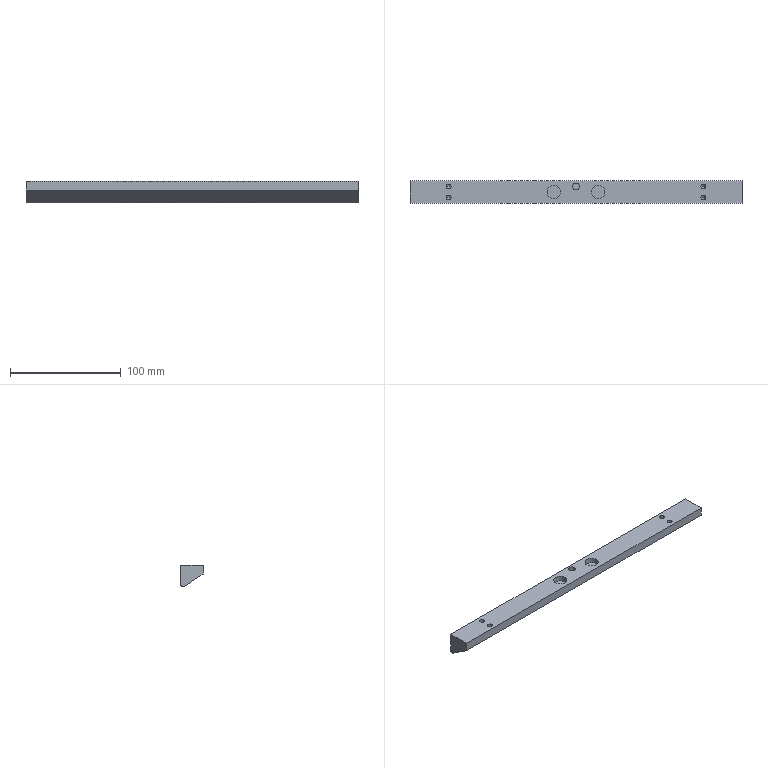Component | SolidWorks | STB-08-007-1 | 1 solid | 32 faces | box 300 x 20 x 19.6 mm | volume 85249 mm3 | cylinder 15 | plane 9 | cone 8 | commonest cylinder face diameters 4.2 x8 12 x4 6.2 x2 4 x1 | material Brass
STEP:
#1=CARTESIAN_POINT('',(-3.579,4.331,-1.417));
#2=VERTEX_POINT('',#1);
#3=CARTESIAN_POINT('',(-3.106,4.331,-1.417));
#4=VERTEX_POINT('',#3);
#5=CARTESIAN_POINT('',(-3.343,4.331,-1.417));
#6=DIRECTION('',(0.,-0.,1.));
#7=DIRECTION('',(1.,0.,0.));
#8=AXIS2_PLACEMENT_3D('',#5,#6,#7);
#9=CIRCLE('',#8,0.2362);
#10=EDGE_CURVE('',#2,#4,#9,.T.);
#11=ORIENTED_EDGE('',*,*,#10,.F.);
#12=CARTESIAN_POINT('',(-3.579,4.331,-1.22));
#13=VERTEX_POINT('',#12);
#14=CARTESIAN_POINT('',(-3.579,4.331,-1.417));
#15=DIRECTION('',(0.,-0.,1.));
#16=VECTOR('',#15,39.37);
#17=LINE('',#14,#16);
#18=EDGE_CURVE('',#2,#13,#17,.T.);
#19=ORIENTED_EDGE('',*,*,#18,.T.);
#20=CARTESIAN_POINT('',(-3.106,4.331,-1.22));
#21=VERTEX_POINT('',#20);
#22=CARTESIAN_POINT('',(-3.343,4.331,-1.22));
#23=DIRECTION('',(0.,-0.,1.));
#24=DIRECTION('',(1.,0.,0.));
#25=AXIS2_PLACEMENT_3D('',#22,#23,#24);
#26=CIRCLE('',#25,0.2362);
#27=EDGE_CURVE('',#13,#21,#26,.T.);
#28=ORIENTED_EDGE('',*,*,#27,.T.);
#29=CARTESIAN_POINT('',(-3.106,4.331,-1.417));
#30=DIRECTION('',(0.,-0.,1.));
#31=VECTOR('',#30,39.37);
#32=LINE('',#29,#31);
#33=EDGE_CURVE('',#4,#21,#32,.T.);
#34=ORIENTED_EDGE('',*,*,#33,.F.);
#35=EDGE_LOOP('',(#11,#19,#28,#34));
#36=FACE_OUTER_BOUND('',#35,.T.);
#37=CARTESIAN_POINT('',(-3.343,4.331,-1.417));
#38=DIRECTION('',(0.,-0.,1.));
#39=DIRECTION('',(1.,0.,0.));
#40=AXIS2_PLACEMENT_3D('',#37,#38,#39);
#41=CYLINDRICAL_SURFACE('',#40,0.2362);
#42=ADVANCED_FACE('',(#36),#41,.F.);
#43=CARTESIAN_POINT('',(-5.154,4.331,-1.417));
#44=VERTEX_POINT('',#43);
#45=CARTESIAN_POINT('',(-4.681,4.331,-1.417));
#46=VERTEX_POINT('',#45);
#47=CARTESIAN_POINT('',(-4.917,4.331,-1.417));
#48=DIRECTION('',(0.,-0.,1.));
#49=DIRECTION('',(1.,0.,0.));
#50=AXIS2_PLACEMENT_3D('',#47,#48,#49);
#51=CIRCLE('',#50,0.2362);
#52=EDGE_CURVE('',#44,#46,#51,.T.);
#53=ORIENTED_EDGE('',*,*,#52,.F.);
#54=CARTESIAN_POINT('',(-5.154,4.331,-1.22));
#55=VERTEX_POINT('',#54);
#56=CARTESIAN_POINT('',(-5.154,4.331,-1.417));
#57=DIRECTION('',(0.,-0.,1.));
#58=VECTOR('',#57,39.37);
#59=LINE('',#56,#58);
#60=EDGE_CURVE('',#44,#55,#59,.T.);
#61=ORIENTED_EDGE('',*,*,#60,.T.);
#62=CARTESIAN_POINT('',(-4.681,4.331,-1.22));
#63=VERTEX_POINT('',#62);
#64=CARTESIAN_POINT('',(-4.917,4.331,-1.22));
#65=DIRECTION('',(0.,-0.,1.));
#66=DIRECTION('',(1.,0.,0.));
#67=AXIS2_PLACEMENT_3D('',#64,#65,#66);
#68=CIRCLE('',#67,0.2362);
#69=EDGE_CURVE('',#55,#63,#68,.T.);
#70=ORIENTED_EDGE('',*,*,#69,.T.);
#71=CARTESIAN_POINT('',(-4.681,4.331,-1.417));
#72=DIRECTION('',(0.,-0.,1.));
#73=VECTOR('',#72,39.37);
#74=LINE('',#71,#73);
#75=EDGE_CURVE('',#46,#63,#74,.T.);
#76=ORIENTED_EDGE('',*,*,#75,.F.);
#77=EDGE_LOOP('',(#53,#61,#70,#76));
#78=FACE_OUTER_BOUND('',#77,.T.);
#79=CARTESIAN_POINT('',(-4.917,4.331,-1.417));
#80=DIRECTION('',(0.,-0.,1.));
#81=DIRECTION('',(1.,0.,0.));
#82=AXIS2_PLACEMENT_3D('',#79,#80,#81);
#83=CYLINDRICAL_SURFACE('',#82,0.2362);
#84=ADVANCED_FACE('',(#78),#83,.F.);
#85=CARTESIAN_POINT('',(-4.13,4.405,-1.417));
#86=VERTEX_POINT('',#85);
#87=CARTESIAN_POINT('',(-4.13,4.65,-1.417));
#88=VERTEX_POINT('',#87);
#89=CARTESIAN_POINT('',(-4.13,4.528,-1.417));
#90=DIRECTION('',(0.,-0.,1.));
#91=DIRECTION('',(0.,1.,0.));
#92=AXIS2_PLACEMENT_3D('',#89,#90,#91);
#93=CIRCLE('',#92,0.122);
#94=EDGE_CURVE('',#86,#88,#93,.T.);
#95=ORIENTED_EDGE('',*,*,#94,.F.);
#96=CARTESIAN_POINT('',(-4.13,4.405,-1.22));
#97=VERTEX_POINT('',#96);
#98=CARTESIAN_POINT('',(-4.13,4.405,-1.417));
#99=DIRECTION('',(0.,-0.,1.));
#100=VECTOR('',#99,39.37);
#101=LINE('',#98,#100);
#102=EDGE_CURVE('',#86,#97,#101,.T.);
#103=ORIENTED_EDGE('',*,*,#102,.T.);
#104=CARTESIAN_POINT('',(-4.13,4.65,-1.22));
#105=VERTEX_POINT('',#104);
#106=CARTESIAN_POINT('',(-4.13,4.528,-1.22));
#107=DIRECTION('',(0.,-0.,1.));
#108=DIRECTION('',(0.,1.,0.));
#109=AXIS2_PLACEMENT_3D('',#106,#107,#108);
#110=CIRCLE('',#109,0.122);
#111=EDGE_CURVE('',#97,#105,#110,.T.);
#112=ORIENTED_EDGE('',*,*,#111,.T.);
#113=CARTESIAN_POINT('',(-4.13,4.65,-1.417));
#114=DIRECTION('',(0.,-0.,1.));
#115=VECTOR('',#114,39.37);
#116=LINE('',#113,#115);
#117=EDGE_CURVE('',#88,#105,#116,.T.);
#118=ORIENTED_EDGE('',*,*,#117,.F.);
#119=EDGE_LOOP('',(#95,#103,#112,#118));
#120=FACE_OUTER_BOUND('',#119,.T.);
#121=CARTESIAN_POINT('',(-4.13,4.528,-1.417));
#122=DIRECTION('',(0.,-0.,1.));
#123=DIRECTION('',(0.,1.,0.));
#124=AXIS2_PLACEMENT_3D('',#121,#122,#123);
#125=CYLINDRICAL_SURFACE('',#124,0.122);
#126=ADVANCED_FACE('',(#120),#125,.F.);
#127=CARTESIAN_POINT('',(-8.74,4.528,-1.575));
#128=VERTEX_POINT('',#127);
#129=CARTESIAN_POINT('',(-8.575,4.528,-1.575));
#130=VERTEX_POINT('',#129);
#131=CARTESIAN_POINT('',(-8.658,4.528,-1.575));
#132=DIRECTION('',(0.,-0.,1.));
#133=DIRECTION('',(1.,0.,0.));
#134=AXIS2_PLACEMENT_3D('',#131,#132,#133);
#135=CIRCLE('',#134,0.08268);
#136=EDGE_CURVE('',#128,#130,#135,.T.);
#137=ORIENTED_EDGE('',*,*,#136,.F.);
#138=CARTESIAN_POINT('',(-8.74,4.528,-1.22));
#139=VERTEX_POINT('',#138);
#140=CARTESIAN_POINT('',(-8.74,4.528,-1.22));
#141=DIRECTION('',(0.,-0.,1.));
#142=VECTOR('',#141,39.37);
#143=LINE('',#140,#142);
#144=EDGE_CURVE('',#128,#139,#143,.T.);
#145=ORIENTED_EDGE('',*,*,#144,.T.);
#146=CARTESIAN_POINT('',(-8.575,4.528,-1.22));
#147=VERTEX_POINT('',#146);
#148=CARTESIAN_POINT('',(-8.658,4.528,-1.22));
#149=DIRECTION('',(0.,-0.,1.));
#150=DIRECTION('',(1.,0.,0.));
#151=AXIS2_PLACEMENT_3D('',#148,#149,#150);
#152=CIRCLE('',#151,0.08268);
#153=EDGE_CURVE('',#139,#147,#152,.T.);
#154=ORIENTED_EDGE('',*,*,#153,.T.);
#155=CARTESIAN_POINT('',(-8.575,4.528,-1.22));
#156=DIRECTION('',(0.,-0.,1.));
#157=VECTOR('',#156,39.37);
#158=LINE('',#155,#157);
#159=EDGE_CURVE('',#130,#147,#158,.T.);
#160=ORIENTED_EDGE('',*,*,#159,.F.);
#161=EDGE_LOOP('',(#137,#145,#154,#160));
#162=FACE_OUTER_BOUND('',#161,.T.);
#163=CARTESIAN_POINT('',(-8.658,4.528,-1.22));
#164=DIRECTION('',(0.,-0.,1.));
#165=DIRECTION('',(1.,0.,0.));
#166=AXIS2_PLACEMENT_3D('',#163,#164,#165);
#167=CYLINDRICAL_SURFACE('',#166,0.08268);
#168=ADVANCED_FACE('',(#162),#167,.F.);
#169=CARTESIAN_POINT('',(-8.658,4.528,-1.624));
#170=VERTEX_POINT('',#169);
#171=CARTESIAN_POINT('',(-8.575,4.528,-1.575));
#172=DIRECTION('',(0.8572,-0.,0.515));
#173=VECTOR('',#172,39.37);
#174=LINE('',#171,#173);
#175=EDGE_CURVE('',#170,#130,#174,.T.);
#176=ORIENTED_EDGE('',*,*,#175,.F.);
#177=CARTESIAN_POINT('',(-8.74,4.528,-1.575));
#178=DIRECTION('',(-0.8572,0.,0.515));
#179=VECTOR('',#178,39.37);
#180=LINE('',#177,#179);
#181=EDGE_CURVE('',#170,#128,#180,.T.);
#182=ORIENTED_EDGE('',*,*,#181,.T.);
#183=ORIENTED_EDGE('',*,*,#136,.T.);
#184=EDGE_LOOP('',(#176,#182,#183));
#185=FACE_OUTER_BOUND('',#184,.T.);
#186=CARTESIAN_POINT('',(-8.658,4.528,-1.575));
#187=DIRECTION('',(0.,-0.,1.));
#188=DIRECTION('',(1.,0.,0.));
#189=AXIS2_PLACEMENT_3D('',#186,#187,#188);
#190=CONICAL_SURFACE('',#189,0.08268,1.03);
#191=ADVANCED_FACE('',(#185),#190,.F.);
#192=CARTESIAN_POINT('',(-8.74,4.134,-1.575));
#193=VERTEX_POINT('',#192);
#194=CARTESIAN_POINT('',(-8.575,4.134,-1.575));
#195=VERTEX_POINT('',#194);
#196=CARTESIAN_POINT('',(-8.658,4.134,-1.575));
#197=DIRECTION('',(0.,-0.,1.));
#198=DIRECTION('',(1.,0.,0.));
#199=AXIS2_PLACEMENT_3D('',#196,#197,#198);
#200=CIRCLE('',#199,0.08268);
#201=EDGE_CURVE('',#193,#195,#200,.T.);
#202=ORIENTED_EDGE('',*,*,#201,.F.);
#203=CARTESIAN_POINT('',(-8.74,4.134,-1.22));
#204=VERTEX_POINT('',#203);
#205=CARTESIAN_POINT('',(-8.74,4.134,-1.22));
#206=DIRECTION('',(0.,-0.,1.));
#207=VECTOR('',#206,39.37);
#208=LINE('',#205,#207);
#209=EDGE_CURVE('',#193,#204,#208,.T.);
#210=ORIENTED_EDGE('',*,*,#209,.T.);
#211=CARTESIAN_POINT('',(-8.575,4.134,-1.22));
#212=VERTEX_POINT('',#211);
#213=CARTESIAN_POINT('',(-8.658,4.134,-1.22));
#214=DIRECTION('',(0.,-0.,1.));
#215=DIRECTION('',(1.,0.,0.));
#216=AXIS2_PLACEMENT_3D('',#213,#214,#215);
#217=CIRCLE('',#216,0.08268);
#218=EDGE_CURVE('',#204,#212,#217,.T.);
#219=ORIENTED_EDGE('',*,*,#218,.T.);
#220=CARTESIAN_POINT('',(-8.575,4.134,-1.22));
#221=DIRECTION('',(0.,-0.,1.));
#222=VECTOR('',#221,39.37);
#223=LINE('',#220,#222);
#224=EDGE_CURVE('',#195,#212,#223,.T.);
#225=ORIENTED_EDGE('',*,*,#224,.F.);
#226=EDGE_LOOP('',(#202,#210,#219,#225));
#227=FACE_OUTER_BOUND('',#226,.T.);
#228=CARTESIAN_POINT('',(-8.658,4.134,-1.22));
#229=DIRECTION('',(0.,-0.,1.));
#230=DIRECTION('',(1.,0.,0.));
#231=AXIS2_PLACEMENT_3D('',#228,#229,#230);
#232=CYLINDRICAL_SURFACE('',#231,0.08268);
#233=ADVANCED_FACE('',(#227),#232,.F.);
#234=CARTESIAN_POINT('',(-8.658,4.134,-1.624));
#235=VERTEX_POINT('',#234);
#236=CARTESIAN_POINT('',(-8.575,4.134,-1.575));
#237=DIRECTION('',(0.8572,-0.,0.515));
#238=VECTOR('',#237,39.37);
#239=LINE('',#236,#238);
#240=EDGE_CURVE('',#235,#195,#239,.T.);
#241=ORIENTED_EDGE('',*,*,#240,.F.);
#242=CARTESIAN_POINT('',(-8.74,4.134,-1.575));
#243=DIRECTION('',(-0.8572,0.,0.515));
#244=VECTOR('',#243,39.37);
#245=LINE('',#242,#244);
#246=EDGE_CURVE('',#235,#193,#245,.T.);
#247=ORIENTED_EDGE('',*,*,#246,.T.);
#248=ORIENTED_EDGE('',*,*,#201,.T.);
#249=EDGE_LOOP('',(#241,#247,#248));
#250=FACE_OUTER_BOUND('',#249,.T.);
#251=CARTESIAN_POINT('',(-8.658,4.134,-1.575));
#252=DIRECTION('',(0.,-0.,1.));
#253=DIRECTION('',(1.,0.,0.));
#254=AXIS2_PLACEMENT_3D('',#251,#252,#253);
#255=CONICAL_SURFACE('',#254,0.08268,1.03);
#256=ADVANCED_FACE('',(#250),#255,.F.);
#257=CARTESIAN_POINT('',(0.3148,4.528,-1.575));
#258=VERTEX_POINT('',#257);
#259=CARTESIAN_POINT('',(0.4802,4.528,-1.575));
#260=VERTEX_POINT('',#259);
#261=CARTESIAN_POINT('',(0.3975,4.528,-1.575));
#262=DIRECTION('',(0.,-0.,1.));
#263=DIRECTION('',(1.,0.,0.));
#264=AXIS2_PLACEMENT_3D('',#261,#262,#263);
#265=CIRCLE('',#264,0.08268);
#266=EDGE_CURVE('',#258,#260,#265,.T.);
#267=ORIENTED_EDGE('',*,*,#266,.F.);
#268=CARTESIAN_POINT('',(0.3148,4.528,-1.22));
#269=VERTEX_POINT('',#268);
#270=CARTESIAN_POINT('',(0.3148,4.528,-1.22));
#271=DIRECTION('',(0.,-0.,1.));
#272=VECTOR('',#271,39.37);
#273=LINE('',#270,#272);
#274=EDGE_CURVE('',#258,#269,#273,.T.);
#275=ORIENTED_EDGE('',*,*,#274,.T.);
#276=CARTESIAN_POINT('',(0.4802,4.528,-1.22));
#277=VERTEX_POINT('',#276);
#278=CARTESIAN_POINT('',(0.3975,4.528,-1.22));
#279=DIRECTION('',(0.,-0.,1.));
#280=DIRECTION('',(1.,0.,0.));
#281=AXIS2_PLACEMENT_3D('',#278,#279,#280);
#282=CIRCLE('',#281,0.08268);
#283=EDGE_CURVE('',#269,#277,#282,.T.);
#284=ORIENTED_EDGE('',*,*,#283,.T.);
#285=CARTESIAN_POINT('',(0.4802,4.528,-1.22));
#286=DIRECTION('',(0.,-0.,1.));
#287=VECTOR('',#286,39.37);
#288=LINE('',#285,#287);
#289=EDGE_CURVE('',#260,#277,#288,.T.);
#290=ORIENTED_EDGE('',*,*,#289,.F.);
#291=EDGE_LOOP('',(#267,#275,#284,#290));
#292=FACE_OUTER_BOUND('',#291,.T.);
#293=CARTESIAN_POINT('',(0.3975,4.528,-1.22));
#294=DIRECTION('',(0.,-0.,1.));
#295=DIRECTION('',(1.,0.,0.));
#296=AXIS2_PLACEMENT_3D('',#293,#294,#295);
#297=CYLINDRICAL_SURFACE('',#296,0.08268);
#298=ADVANCED_FACE('',(#292),#297,.F.);
#299=CARTESIAN_POINT('',(0.3975,4.528,-1.624));
#300=VERTEX_POINT('',#299);
#301=CARTESIAN_POINT('',(0.4802,4.528,-1.575));
#302=DIRECTION('',(0.8572,-0.,0.515));
#303=VECTOR('',#302,39.37);
#304=LINE('',#301,#303);
#305=EDGE_CURVE('',#300,#260,#304,.T.);
#306=ORIENTED_EDGE('',*,*,#305,.F.);
#307=CARTESIAN_POINT('',(0.3148,4.528,-1.575));
#308=DIRECTION('',(-0.8572,0.,0.515));
#309=VECTOR('',#308,39.37);
#310=LINE('',#307,#309);
#311=EDGE_CURVE('',#300,#258,#310,.T.);
#312=ORIENTED_EDGE('',*,*,#311,.T.);
#313=ORIENTED_EDGE('',*,*,#266,.T.);
#314=EDGE_LOOP('',(#306,#312,#313));
#315=FACE_OUTER_BOUND('',#314,.T.);
#316=CARTESIAN_POINT('',(0.3975,4.528,-1.575));
#317=DIRECTION('',(0.,-0.,1.));
#318=DIRECTION('',(1.,0.,0.));
#319=AXIS2_PLACEMENT_3D('',#316,#317,#318);
#320=CONICAL_SURFACE('',#319,0.08268,1.03);
#321=ADVANCED_FACE('',(#315),#320,.F.);
#322=CARTESIAN_POINT('',(0.3148,4.134,-1.575));
#323=VERTEX_POINT('',#322);
#324=CARTESIAN_POINT('',(0.4802,4.134,-1.575));
#325=VERTEX_POINT('',#324);
#326=CARTESIAN_POINT('',(0.3975,4.134,-1.575));
#327=DIRECTION('',(0.,-0.,1.));
#328=DIRECTION('',(1.,0.,0.));
#329=AXIS2_PLACEMENT_3D('',#326,#327,#328);
#330=CIRCLE('',#329,0.08268);
#331=EDGE_CURVE('',#323,#325,#330,.T.);
#332=ORIENTED_EDGE('',*,*,#331,.F.);
#333=CARTESIAN_POINT('',(0.3148,4.134,-1.22));
#334=VERTEX_POINT('',#333);
#335=CARTESIAN_POINT('',(0.3148,4.134,-1.22));
#336=DIRECTION('',(0.,-0.,1.));
#337=VECTOR('',#336,39.37);
#338=LINE('',#335,#337);
#339=EDGE_CURVE('',#323,#334,#338,.T.);
#340=ORIENTED_EDGE('',*,*,#339,.T.);
#341=CARTESIAN_POINT('',(0.4802,4.134,-1.22));
#342=VERTEX_POINT('',#341);
#343=CARTESIAN_POINT('',(0.3975,4.134,-1.22));
#344=DIRECTION('',(0.,-0.,1.));
#345=DIRECTION('',(1.,0.,0.));
#346=AXIS2_PLACEMENT_3D('',#343,#344,#345);
#347=CIRCLE('',#346,0.08268);
#348=EDGE_CURVE('',#334,#342,#347,.T.);
#349=ORIENTED_EDGE('',*,*,#348,.T.);
#350=CARTESIAN_POINT('',(0.4802,4.134,-1.22));
#351=DIRECTION('',(0.,-0.,1.));
#352=VECTOR('',#351,39.37);
#353=LINE('',#350,#352);
#354=EDGE_CURVE('',#325,#342,#353,.T.);
#355=ORIENTED_EDGE('',*,*,#354,.F.);
#356=EDGE_LOOP('',(#332,#340,#349,#355));
#357=FACE_OUTER_BOUND('',#356,.T.);
#358=CARTESIAN_POINT('',(0.3975,4.134,-1.22));
#359=DIRECTION('',(0.,-0.,1.));
#360=DIRECTION('',(1.,0.,0.));
#361=AXIS2_PLACEMENT_3D('',#358,#359,#360);
#362=CYLINDRICAL_SURFACE('',#361,0.08268);
#363=ADVANCED_FACE('',(#357),#362,.F.);
#364=CARTESIAN_POINT('',(0.3975,4.134,-1.624));
#365=VERTEX_POINT('',#364);
#366=CARTESIAN_POINT('',(0.4802,4.134,-1.575));
#367=DIRECTION('',(0.8572,-0.,0.515));
#368=VECTOR('',#367,39.37);
#369=LINE('',#366,#368);
#370=EDGE_CURVE('',#365,#325,#369,.T.);
#371=ORIENTED_EDGE('',*,*,#370,.F.);
#372=CARTESIAN_POINT('',(0.3148,4.134,-1.575));
#373=DIRECTION('',(-0.8572,0.,0.515));
#374=VECTOR('',#373,39.37);
#375=LINE('',#372,#374);
#376=EDGE_CURVE('',#365,#323,#375,.T.);
#377=ORIENTED_EDGE('',*,*,#376,.T.);
#378=ORIENTED_EDGE('',*,*,#331,.T.);
#379=EDGE_LOOP('',(#371,#377,#378));
#380=FACE_OUTER_BOUND('',#379,.T.);
#381=CARTESIAN_POINT('',(0.3975,4.134,-1.575));
#382=DIRECTION('',(0.,-0.,1.));
#383=DIRECTION('',(1.,0.,0.));
#384=AXIS2_PLACEMENT_3D('',#381,#382,#383);
#385=CONICAL_SURFACE('',#384,0.08268,1.03);
#386=ADVANCED_FACE('',(#380),#385,.F.);
#387=CARTESIAN_POINT('',(-10.036,3.937,-1.535));
#388=VERTEX_POINT('',#387);
#389=CARTESIAN_POINT('',(-10.036,3.937,-1.22));
#390=VERTEX_POINT('',#389);
#391=CARTESIAN_POINT('',(-10.036,3.937,-2.008));
#392=DIRECTION('',(0.,-0.,1.));
#393=VECTOR('',#392,39.37);
#394=LINE('',#391,#393);
#395=EDGE_CURVE('',#388,#390,#394,.T.);
#396=ORIENTED_EDGE('',*,*,#395,.F.);
#397=CARTESIAN_POINT('',(1.775,3.937,-1.535));
#398=VERTEX_POINT('',#397);
#399=CARTESIAN_POINT('',(1.775,3.937,-1.535));
#400=DIRECTION('',(-1.,0.,0.));
#401=VECTOR('',#400,39.37);
#402=LINE('',#399,#401);
#403=EDGE_CURVE('',#398,#388,#402,.T.);
#404=ORIENTED_EDGE('',*,*,#403,.F.);
#405=CARTESIAN_POINT('',(1.775,3.937,-1.22));
#406=VERTEX_POINT('',#405);
#407=CARTESIAN_POINT('',(1.775,3.937,-2.008));
#408=DIRECTION('',(0.,-0.,1.));
#409=VECTOR('',#408,39.37);
#410=LINE('',#407,#409);
#411=EDGE_CURVE('',#398,#406,#410,.T.);
#412=ORIENTED_EDGE('',*,*,#411,.T.);
#413=CARTESIAN_POINT('',(-10.036,3.937,-1.22));
#414=DIRECTION('',(1.,-0.,-0.));
#415=VECTOR('',#414,39.37);
#416=LINE('',#413,#415);
#417=EDGE_CURVE('',#390,#406,#416,.T.);
#418=ORIENTED_EDGE('',*,*,#417,.F.);
#419=EDGE_LOOP('',(#396,#404,#412,#418));
#420=FACE_OUTER_BOUND('',#419,.T.);
#421=CARTESIAN_POINT('',(-10.036,3.937,-2.008));
#422=DIRECTION('',(0.,1.,0.));
#423=DIRECTION('',(-1.,0.,0.));
#424=AXIS2_PLACEMENT_3D('',#421,#422,#423);
#425=PLANE('',#424);
#426=ADVANCED_FACE('',(#420),#425,.F.);
#427=CARTESIAN_POINT('',(-3.343,4.331,-1.22));
#428=DIRECTION('',(0.,-0.,1.));
#429=DIRECTION('',(1.,0.,0.));
#430=AXIS2_PLACEMENT_3D('',#427,#428,#429);
#431=CIRCLE('',#430,0.2362);
#432=EDGE_CURVE('',#21,#13,#431,.T.);
#433=ORIENTED_EDGE('',*,*,#432,.F.);
#434=ORIENTED_EDGE('',*,*,#27,.F.);
#435=EDGE_LOOP('',(#433,#434));
#436=FACE_BOUND('',#435,.T.);
#437=CARTESIAN_POINT('',(-4.917,4.331,-1.22));
#438=DIRECTION('',(0.,-0.,1.));
#439=DIRECTION('',(1.,0.,0.));
#440=AXIS2_PLACEMENT_3D('',#437,#438,#439);
#441=CIRCLE('',#440,0.2362);
#442=EDGE_CURVE('',#63,#55,#441,.T.);
#443=ORIENTED_EDGE('',*,*,#442,.F.);
#444=ORIENTED_EDGE('',*,*,#69,.F.);
#445=EDGE_LOOP('',(#443,#444));
#446=FACE_BOUND('',#445,.T.);
#447=CARTESIAN_POINT('',(-4.13,4.528,-1.22));
#448=DIRECTION('',(0.,-0.,1.));
#449=DIRECTION('',(0.,1.,0.));
#450=AXIS2_PLACEMENT_3D('',#447,#448,#449);
#451=CIRCLE('',#450,0.122);
#452=EDGE_CURVE('',#105,#97,#451,.T.);
#453=ORIENTED_EDGE('',*,*,#452,.F.);
#454=ORIENTED_EDGE('',*,*,#111,.F.);
#455=EDGE_LOOP('',(#453,#454));
#456=FACE_BOUND('',#455,.T.);
#457=CARTESIAN_POINT('',(-8.658,4.528,-1.22));
#458=DIRECTION('',(0.,-0.,1.));
#459=DIRECTION('',(1.,0.,0.));
#460=AXIS2_PLACEMENT_3D('',#457,#458,#459);
#461=CIRCLE('',#460,0.08268);
#462=EDGE_CURVE('',#147,#139,#461,.T.);
#463=ORIENTED_EDGE('',*,*,#462,.F.);
#464=ORIENTED_EDGE('',*,*,#153,.F.);
#465=EDGE_LOOP('',(#463,#464));
#466=FACE_BOUND('',#465,.T.);
#467=CARTESIAN_POINT('',(-8.658,4.134,-1.22));
#468=DIRECTION('',(0.,-0.,1.));
#469=DIRECTION('',(1.,0.,0.));
#470=AXIS2_PLACEMENT_3D('',#467,#468,#469);
#471=CIRCLE('',#470,0.08268);
#472=EDGE_CURVE('',#212,#204,#471,.T.);
#473=ORIENTED_EDGE('',*,*,#472,.F.);
#474=ORIENTED_EDGE('',*,*,#218,.F.);
#475=EDGE_LOOP('',(#473,#474));
#476=FACE_BOUND('',#475,.T.);
#477=CARTESIAN_POINT('',(0.3975,4.528,-1.22));
#478=DIRECTION('',(0.,-0.,1.));
#479=DIRECTION('',(1.,0.,0.));
#480=AXIS2_PLACEMENT_3D('',#477,#478,#479);
#481=CIRCLE('',#480,0.08268);
#482=EDGE_CURVE('',#277,#269,#481,.T.);
#483=ORIENTED_EDGE('',*,*,#482,.F.);
#484=ORIENTED_EDGE('',*,*,#283,.F.);
#485=EDGE_LOOP('',(#483,#484));
#486=FACE_BOUND('',#485,.T.);
#487=CARTESIAN_POINT('',(0.3975,4.134,-1.22));
#488=DIRECTION('',(0.,-0.,1.));
#489=DIRECTION('',(1.,0.,0.));
#490=AXIS2_PLACEMENT_3D('',#487,#488,#489);
#491=CIRCLE('',#490,0.08268);
#492=EDGE_CURVE('',#342,#334,#491,.T.);
#493=ORIENTED_EDGE('',*,*,#492,.F.);
#494=ORIENTED_EDGE('',*,*,#348,.F.);
#495=EDGE_LOOP('',(#493,#494));
#496=FACE_BOUND('',#495,.T.);
#497=CARTESIAN_POINT('',(1.775,4.724,-1.22));
#498=VERTEX_POINT('',#497);
#499=CARTESIAN_POINT('',(1.775,4.724,-1.22));
#500=DIRECTION('',(0.,1.,0.));
#501=VECTOR('',#500,39.37);
#502=LINE('',#499,#501);
#503=EDGE_CURVE('',#406,#498,#502,.T.);
#504=ORIENTED_EDGE('',*,*,#503,.T.);
#505=CARTESIAN_POINT('',(-10.036,4.724,-1.22));
#506=VERTEX_POINT('',#505);
#507=CARTESIAN_POINT('',(-10.036,4.724,-1.22));
#508=DIRECTION('',(1.,-0.,-0.));
#509=VECTOR('',#508,39.37);
#510=LINE('',#507,#509);
#511=EDGE_CURVE('',#506,#498,#510,.T.);
#512=ORIENTED_EDGE('',*,*,#511,.F.);
#513=CARTESIAN_POINT('',(-10.036,4.724,-1.22));
#514=DIRECTION('',(0.,1.,0.));
#515=VECTOR('',#514,39.37);
#516=LINE('',#513,#515);
#517=EDGE_CURVE('',#390,#506,#516,.T.);
#518=ORIENTED_EDGE('',*,*,#517,.F.);
#519=ORIENTED_EDGE('',*,*,#417,.T.);
#520=EDGE_LOOP('',(#504,#512,#518,#519));
#521=FACE_OUTER_BOUND('',#520,.T.);
#522=CARTESIAN_POINT('',(-10.036,4.724,-1.22));
#523=DIRECTION('',(-0.,0.,-1.));
#524=DIRECTION('',(-1.,0.,0.));
#525=AXIS2_PLACEMENT_3D('',#522,#523,#524);
#526=PLANE('',#525);
#527=ADVANCED_FACE('',(#436,#446,#456,#466,#476,#486,#496,#521),#526,.F.);
#528=CARTESIAN_POINT('',(1.775,4.724,-1.913));
#529=VERTEX_POINT('',#528);
#530=CARTESIAN_POINT('',(1.775,4.724,-2.008));
#531=DIRECTION('',(-0.,0.,-1.));
#532=VECTOR('',#531,39.37);
#533=LINE('',#530,#532);
#534=EDGE_CURVE('',#498,#529,#533,.T.);
#535=ORIENTED_EDGE('',*,*,#534,.T.);
#536=CARTESIAN_POINT('',(-10.036,4.724,-1.913));
#537=VERTEX_POINT('',#536);
#538=CARTESIAN_POINT('',(-10.036,4.724,-1.913));
#539=DIRECTION('',(-1.,0.,0.));
#540=VECTOR('',#539,39.37);
#541=LINE('',#538,#540);
#542=EDGE_CURVE('',#529,#537,#541,.T.);
#543=ORIENTED_EDGE('',*,*,#542,.T.);
#544=CARTESIAN_POINT('',(-10.036,4.724,-2.008));
#545=DIRECTION('',(-0.,0.,-1.));
#546=VECTOR('',#545,39.37);
#547=LINE('',#544,#546);
#548=EDGE_CURVE('',#506,#537,#547,.T.);
#549=ORIENTED_EDGE('',*,*,#548,.F.);
#550=ORIENTED_EDGE('',*,*,#511,.T.);
#551=EDGE_LOOP('',(#535,#543,#549,#550));
#552=FACE_OUTER_BOUND('',#551,.T.);
#553=CARTESIAN_POINT('',(-10.036,4.724,-2.008));
#554=DIRECTION('',(-0.,-1.,-0.));
#555=DIRECTION('',(1.,-0.,-0.));
#556=AXIS2_PLACEMENT_3D('',#553,#554,#555);
#557=PLANE('',#556);
#558=ADVANCED_FACE('',(#552),#557,.F.);
#559=ORIENTED_EDGE('',*,*,#548,.T.);
#560=CARTESIAN_POINT('',(-10.036,4.602,-1.979));
#561=VERTEX_POINT('',#560);
#562=CARTESIAN_POINT('',(-10.036,4.646,-1.913));
#563=DIRECTION('',(-1.,0.,0.));
#564=DIRECTION('',(0.,0.,1.));
#565=AXIS2_PLACEMENT_3D('',#562,#563,#564);
#566=CIRCLE('',#565,0.07874);
#567=EDGE_CURVE('',#537,#561,#566,.T.);
#568=ORIENTED_EDGE('',*,*,#567,.T.);
#569=CARTESIAN_POINT('',(-10.036,4.646,-2.008));
#570=DIRECTION('',(-0.,0.8321,-0.5547));
#571=VECTOR('',#570,39.37);
#572=LINE('',#569,#571);
#573=EDGE_CURVE('',#388,#561,#572,.T.);
#574=ORIENTED_EDGE('',*,*,#573,.F.);
#575=ORIENTED_EDGE('',*,*,#395,.T.);
#576=ORIENTED_EDGE('',*,*,#517,.T.);
#577=EDGE_LOOP('',(#559,#568,#574,#575,#576));
#578=FACE_OUTER_BOUND('',#577,.T.);
#579=CARTESIAN_POINT('',(-10.036,3.937,-2.008));
#580=DIRECTION('',(-1.,0.,0.));
#581=DIRECTION('',(0.,-0.,1.));
#582=AXIS2_PLACEMENT_3D('',#579,#580,#581);
#583=PLANE('',#582);
#584=ADVANCED_FACE('',(#578),#583,.T.);
#585=CARTESIAN_POINT('',(1.775,4.602,-1.979));
#586=VERTEX_POINT('',#585);
#587=CARTESIAN_POINT('',(1.775,4.646,-2.008));
#588=DIRECTION('',(0.,-0.8321,0.5547));
#589=VECTOR('',#588,39.37);
#590=LINE('',#587,#589);
#591=EDGE_CURVE('',#586,#398,#590,.T.);
#592=ORIENTED_EDGE('',*,*,#591,.F.);
#593=CARTESIAN_POINT('',(1.775,4.646,-1.913));
#594=DIRECTION('',(1.,-0.,-0.));
#595=DIRECTION('',(0.,-0.,1.));
#596=AXIS2_PLACEMENT_3D('',#593,#594,#595);
#597=CIRCLE('',#596,0.07874);
#598=EDGE_CURVE('',#586,#529,#597,.T.);
#599=ORIENTED_EDGE('',*,*,#598,.T.);
#600=ORIENTED_EDGE('',*,*,#534,.F.);
#601=ORIENTED_EDGE('',*,*,#503,.F.);
#602=ORIENTED_EDGE('',*,*,#411,.F.);
#603=EDGE_LOOP('',(#592,#599,#600,#601,#602));
#604=FACE_OUTER_BOUND('',#603,.T.);
#605=CARTESIAN_POINT('',(1.775,3.937,-2.008));
#606=DIRECTION('',(-1.,0.,0.));
#607=DIRECTION('',(0.,-0.,1.));
#608=AXIS2_PLACEMENT_3D('',#605,#606,#607);
#609=PLANE('',#608);
#610=ADVANCED_FACE('',(#604),#609,.F.);
#611=ORIENTED_EDGE('',*,*,#573,.T.);
#612=CARTESIAN_POINT('',(1.775,4.602,-1.979));
#613=DIRECTION('',(1.,-0.,-0.));
#614=VECTOR('',#613,39.37);
#615=LINE('',#612,#614);
#616=EDGE_CURVE('',#561,#586,#615,.T.);
#617=ORIENTED_EDGE('',*,*,#616,.T.);
#618=ORIENTED_EDGE('',*,*,#591,.T.);
#619=ORIENTED_EDGE('',*,*,#403,.T.);
#620=EDGE_LOOP('',(#611,#617,#618,#619));
#621=FACE_OUTER_BOUND('',#620,.T.);
#622=CARTESIAN_POINT('',(1.775,4.646,-2.008));
#623=DIRECTION('',(0.,0.5547,0.8321));
#624=DIRECTION('',(-0.,0.8321,-0.5547));
#625=AXIS2_PLACEMENT_3D('',#622,#623,#624);
#626=PLANE('',#625);
#627=ADVANCED_FACE('',(#621),#626,.F.);
#628=ORIENTED_EDGE('',*,*,#376,.F.);
#629=ORIENTED_EDGE('',*,*,#370,.T.);
#630=CARTESIAN_POINT('',(0.3975,4.134,-1.575));
#631=DIRECTION('',(0.,-0.,1.));
#632=DIRECTION('',(1.,0.,0.));
#633=AXIS2_PLACEMENT_3D('',#630,#631,#632);
#634=CIRCLE('',#633,0.08268);
#635=EDGE_CURVE('',#325,#323,#634,.T.);
#636=ORIENTED_EDGE('',*,*,#635,.T.);
#637=EDGE_LOOP('',(#628,#629,#636));
#638=FACE_OUTER_BOUND('',#637,.T.);
#639=CARTESIAN_POINT('',(0.3975,4.134,-1.575));
#640=DIRECTION('',(0.,-0.,1.));
#641=DIRECTION('',(1.,0.,0.));
#642=AXIS2_PLACEMENT_3D('',#639,#640,#641);
#643=CONICAL_SURFACE('',#642,0.08268,1.03);
#644=ADVANCED_FACE('',(#638),#643,.F.);
#645=ORIENTED_EDGE('',*,*,#339,.F.);
#646=ORIENTED_EDGE('',*,*,#635,.F.);
#647=ORIENTED_EDGE('',*,*,#354,.T.);
#648=ORIENTED_EDGE('',*,*,#492,.T.);
#649=EDGE_LOOP('',(#645,#646,#647,#648));
#650=FACE_OUTER_BOUND('',#649,.T.);
#651=CARTESIAN_POINT('',(0.3975,4.134,-1.22));
#652=DIRECTION('',(0.,-0.,1.));
#653=DIRECTION('',(1.,0.,0.));
#654=AXIS2_PLACEMENT_3D('',#651,#652,#653);
#655=CYLINDRICAL_SURFACE('',#654,0.08268);
#656=ADVANCED_FACE('',(#650),#655,.F.);
#657=ORIENTED_EDGE('',*,*,#311,.F.);
#658=ORIENTED_EDGE('',*,*,#305,.T.);
#659=CARTESIAN_POINT('',(0.3975,4.528,-1.575));
#660=DIRECTION('',(0.,-0.,1.));
#661=DIRECTION('',(1.,0.,0.));
#662=AXIS2_PLACEMENT_3D('',#659,#660,#661);
#663=CIRCLE('',#662,0.08268);
#664=EDGE_CURVE('',#260,#258,#663,.T.);
#665=ORIENTED_EDGE('',*,*,#664,.T.);
#666=EDGE_LOOP('',(#657,#658,#665));
#667=FACE_OUTER_BOUND('',#666,.T.);
#668=CARTESIAN_POINT('',(0.3975,4.528,-1.575));
#669=DIRECTION('',(0.,-0.,1.));
#670=DIRECTION('',(1.,0.,0.));
#671=AXIS2_PLACEMENT_3D('',#668,#669,#670);
#672=CONICAL_SURFACE('',#671,0.08268,1.03);
#673=ADVANCED_FACE('',(#667),#672,.F.);
#674=ORIENTED_EDGE('',*,*,#274,.F.);
#675=ORIENTED_EDGE('',*,*,#664,.F.);
#676=ORIENTED_EDGE('',*,*,#289,.T.);
#677=ORIENTED_EDGE('',*,*,#482,.T.);
#678=EDGE_LOOP('',(#674,#675,#676,#677));
#679=FACE_OUTER_BOUND('',#678,.T.);
#680=CARTESIAN_POINT('',(0.3975,4.528,-1.22));
#681=DIRECTION('',(0.,-0.,1.));
#682=DIRECTION('',(1.,0.,0.));
#683=AXIS2_PLACEMENT_3D('',#680,#681,#682);
#684=CYLINDRICAL_SURFACE('',#683,0.08268);
#685=ADVANCED_FACE('',(#679),#684,.F.);
#686=ORIENTED_EDGE('',*,*,#246,.F.);
#687=ORIENTED_EDGE('',*,*,#240,.T.);
#688=CARTESIAN_POINT('',(-8.658,4.134,-1.575));
#689=DIRECTION('',(0.,-0.,1.));
#690=DIRECTION('',(1.,0.,0.));
#691=AXIS2_PLACEMENT_3D('',#688,#689,#690);
#692=CIRCLE('',#691,0.08268);
#693=EDGE_CURVE('',#195,#193,#692,.T.);
#694=ORIENTED_EDGE('',*,*,#693,.T.);
#695=EDGE_LOOP('',(#686,#687,#694));
#696=FACE_OUTER_BOUND('',#695,.T.);
#697=CARTESIAN_POINT('',(-8.658,4.134,-1.575));
#698=DIRECTION('',(0.,-0.,1.));
#699=DIRECTION('',(1.,0.,0.));
#700=AXIS2_PLACEMENT_3D('',#697,#698,#699);
#701=CONICAL_SURFACE('',#700,0.08268,1.03);
#702=ADVANCED_FACE('',(#696),#701,.F.);
#703=ORIENTED_EDGE('',*,*,#209,.F.);
#704=ORIENTED_EDGE('',*,*,#693,.F.);
#705=ORIENTED_EDGE('',*,*,#224,.T.);
#706=ORIENTED_EDGE('',*,*,#472,.T.);
#707=EDGE_LOOP('',(#703,#704,#705,#706));
#708=FACE_OUTER_BOUND('',#707,.T.);
#709=CARTESIAN_POINT('',(-8.658,4.134,-1.22));
#710=DIRECTION('',(0.,-0.,1.));
#711=DIRECTION('',(1.,0.,0.));
#712=AXIS2_PLACEMENT_3D('',#709,#710,#711);
#713=CYLINDRICAL_SURFACE('',#712,0.08268);
#714=ADVANCED_FACE('',(#708),#713,.F.);
#715=ORIENTED_EDGE('',*,*,#181,.F.);
#716=ORIENTED_EDGE('',*,*,#175,.T.);
#717=CARTESIAN_POINT('',(-8.658,4.528,-1.575));
#718=DIRECTION('',(0.,-0.,1.));
#719=DIRECTION('',(1.,0.,0.));
#720=AXIS2_PLACEMENT_3D('',#717,#718,#719);
#721=CIRCLE('',#720,0.08268);
#722=EDGE_CURVE('',#130,#128,#721,.T.);
#723=ORIENTED_EDGE('',*,*,#722,.T.);
#724=EDGE_LOOP('',(#715,#716,#723));
#725=FACE_OUTER_BOUND('',#724,.T.);
#726=CARTESIAN_POINT('',(-8.658,4.528,-1.575));
#727=DIRECTION('',(0.,-0.,1.));
#728=DIRECTION('',(1.,0.,0.));
#729=AXIS2_PLACEMENT_3D('',#726,#727,#728);
#730=CONICAL_SURFACE('',#729,0.08268,1.03);
#731=ADVANCED_FACE('',(#725),#730,.F.);
#732=ORIENTED_EDGE('',*,*,#144,.F.);
#733=ORIENTED_EDGE('',*,*,#722,.F.);
#734=ORIENTED_EDGE('',*,*,#159,.T.);
#735=ORIENTED_EDGE('',*,*,#462,.T.);
#736=EDGE_LOOP('',(#732,#733,#734,#735));
#737=FACE_OUTER_BOUND('',#736,.T.);
#738=CARTESIAN_POINT('',(-8.658,4.528,-1.22));
#739=DIRECTION('',(0.,-0.,1.));
#740=DIRECTION('',(1.,0.,0.));
#741=AXIS2_PLACEMENT_3D('',#738,#739,#740);
#742=CYLINDRICAL_SURFACE('',#741,0.08268);
#743=ADVANCED_FACE('',(#737),#742,.F.);
#744=ORIENTED_EDGE('',*,*,#102,.F.);
#745=CARTESIAN_POINT('',(-4.13,4.528,-1.417));
#746=DIRECTION('',(0.,-0.,1.));
#747=DIRECTION('',(0.,1.,0.));
#748=AXIS2_PLACEMENT_3D('',#745,#746,#747);
#749=CIRCLE('',#748,0.122);
#750=EDGE_CURVE('',#88,#86,#749,.T.);
#751=ORIENTED_EDGE('',*,*,#750,.F.);
#752=ORIENTED_EDGE('',*,*,#117,.T.);
#753=ORIENTED_EDGE('',*,*,#452,.T.);
#754=EDGE_LOOP('',(#744,#751,#752,#753));
#755=FACE_OUTER_BOUND('',#754,.T.);
#756=CARTESIAN_POINT('',(-4.13,4.528,-1.417));
#757=DIRECTION('',(0.,-0.,1.));
#758=DIRECTION('',(0.,1.,0.));
#759=AXIS2_PLACEMENT_3D('',#756,#757,#758);
#760=CYLINDRICAL_SURFACE('',#759,0.122);
#761=ADVANCED_FACE('',(#755),#760,.F.);
#762=ORIENTED_EDGE('',*,*,#750,.T.);
#763=ORIENTED_EDGE('',*,*,#94,.T.);
#764=EDGE_LOOP('',(#762,#763));
#765=FACE_OUTER_BOUND('',#764,.T.);
#766=CARTESIAN_POINT('',(-4.13,4.528,-1.417));
#767=DIRECTION('',(0.,-0.,1.));
#768=DIRECTION('',(-0.,1.,0.));
#769=AXIS2_PLACEMENT_3D('',#766,#767,#768);
#770=PLANE('',#769);
#771=ADVANCED_FACE('',(#765),#770,.T.);
#772=ORIENTED_EDGE('',*,*,#60,.F.);
#773=CARTESIAN_POINT('',(-4.917,4.331,-1.417));
#774=DIRECTION('',(0.,-0.,1.));
#775=DIRECTION('',(1.,0.,0.));
#776=AXIS2_PLACEMENT_3D('',#773,#774,#775);
#777=CIRCLE('',#776,0.2362);
#778=EDGE_CURVE('',#46,#44,#777,.T.);
#779=ORIENTED_EDGE('',*,*,#778,.F.);
#780=ORIENTED_EDGE('',*,*,#75,.T.);
#781=ORIENTED_EDGE('',*,*,#442,.T.);
#782=EDGE_LOOP('',(#772,#779,#780,#781));
#783=FACE_OUTER_BOUND('',#782,.T.);
#784=CARTESIAN_POINT('',(-4.917,4.331,-1.417));
#785=DIRECTION('',(0.,-0.,1.));
#786=DIRECTION('',(1.,0.,0.));
#787=AXIS2_PLACEMENT_3D('',#784,#785,#786);
#788=CYLINDRICAL_SURFACE('',#787,0.2362);
#789=ADVANCED_FACE('',(#783),#788,.F.);
#790=ORIENTED_EDGE('',*,*,#778,.T.);
#791=ORIENTED_EDGE('',*,*,#52,.T.);
#792=EDGE_LOOP('',(#790,#791));
#793=FACE_OUTER_BOUND('',#792,.T.);
#794=CARTESIAN_POINT('',(-4.917,4.331,-1.417));
#795=DIRECTION('',(0.,-0.,1.));
#796=DIRECTION('',(1.,-0.,-0.));
#797=AXIS2_PLACEMENT_3D('',#794,#795,#796);
#798=PLANE('',#797);
#799=ADVANCED_FACE('',(#793),#798,.T.);
#800=ORIENTED_EDGE('',*,*,#18,.F.);
#801=CARTESIAN_POINT('',(-3.343,4.331,-1.417));
#802=DIRECTION('',(0.,-0.,1.));
#803=DIRECTION('',(1.,0.,0.));
#804=AXIS2_PLACEMENT_3D('',#801,#802,#803);
#805=CIRCLE('',#804,0.2362);
#806=EDGE_CURVE('',#4,#2,#805,.T.);
#807=ORIENTED_EDGE('',*,*,#806,.F.);
#808=ORIENTED_EDGE('',*,*,#33,.T.);
#809=ORIENTED_EDGE('',*,*,#432,.T.);
#810=EDGE_LOOP('',(#800,#807,#808,#809));
#811=FACE_OUTER_BOUND('',#810,.T.);
#812=CARTESIAN_POINT('',(-3.343,4.331,-1.417));
#813=DIRECTION('',(0.,-0.,1.));
#814=DIRECTION('',(1.,0.,0.));
#815=AXIS2_PLACEMENT_3D('',#812,#813,#814);
#816=CYLINDRICAL_SURFACE('',#815,0.2362);
#817=ADVANCED_FACE('',(#811),#816,.F.);
#818=ORIENTED_EDGE('',*,*,#806,.T.);
#819=ORIENTED_EDGE('',*,*,#10,.T.);
#820=EDGE_LOOP('',(#818,#819));
#821=FACE_OUTER_BOUND('',#820,.T.);
#822=CARTESIAN_POINT('',(-3.343,4.331,-1.417));
#823=DIRECTION('',(0.,-0.,1.));
#824=DIRECTION('',(1.,-0.,-0.));
#825=AXIS2_PLACEMENT_3D('',#822,#823,#824);
#826=PLANE('',#825);
#827=ADVANCED_FACE('',(#821),#826,.T.);
#828=ORIENTED_EDGE('',*,*,#598,.F.);
#829=ORIENTED_EDGE('',*,*,#616,.F.);
#830=ORIENTED_EDGE('',*,*,#567,.F.);
#831=ORIENTED_EDGE('',*,*,#542,.F.);
#832=EDGE_LOOP('',(#828,#829,#830,#831));
#833=FACE_OUTER_BOUND('',#832,.T.);
#834=CARTESIAN_POINT('',(-10.036,4.646,-1.913));
#835=DIRECTION('',(-1.,0.,0.));
#836=DIRECTION('',(0.,0.,1.));
#837=AXIS2_PLACEMENT_3D('',#834,#835,#836);
#838=CYLINDRICAL_SURFACE('',#837,0.07874);
#839=ADVANCED_FACE('',(#833),#838,.T.);
#840=CLOSED_SHELL('',(#42,#84,#126,#168,#191,#233,#256,#298,#321,#363,#386,#426,#527,#558,#584,#610,#627,#644,#656,#673,#685,#702,#714,#731,#743,#761,#771,#789,#799,#817,#827,#839));
#841=MANIFOLD_SOLID_BREP('',#840);
#842=CARTESIAN_POINT('',(0.,0.,0.));
#843=DIRECTION('',(0.,0.,1.));
#844=DIRECTION('',(1.,0.,0.));
#845=AXIS2_PLACEMENT_3D('',#842,#843,#844);
#846=(LENGTH_UNIT()NAMED_UNIT(*)SI_UNIT($,.METRE.));
#847=LENGTH_MEASURE_WITH_UNIT(LENGTH_MEASURE(0.0254),#846);
#848=DIMENSIONAL_EXPONENTS(1.,0.,0.,0.,0.,0.,0.);
#849=(CONVERSION_BASED_UNIT('',#847)LENGTH_UNIT()NAMED_UNIT(#848));
#850=UNCERTAINTY_MEASURE_WITH_UNIT(LENGTH_MEASURE(0.00001),#849,'','');
#851=(NAMED_UNIT(*)PLANE_ANGLE_UNIT()SI_UNIT($,.RADIAN.));
#852=(NAMED_UNIT(*)SI_UNIT($,.STERADIAN.)SOLID_ANGLE_UNIT());
#853=(GEOMETRIC_REPRESENTATION_CONTEXT(3)GLOBAL_UNCERTAINTY_ASSIGNED_CONTEXT((#850))GLOBAL_UNIT_ASSIGNED_CONTEXT((#849,#851,#852))REPRESENTATION_CONTEXT('',''));
#854=ADVANCED_BREP_SHAPE_REPRESENTATION('',(#841,#845),#853);
#855=COLOUR_RGB('',0.7922,0.8196,0.9333);
#856=FILL_AREA_STYLE_COLOUR('',#855);
#857=FILL_AREA_STYLE('',(#856));
#858=SURFACE_STYLE_FILL_AREA(#857);
#859=SURFACE_SIDE_STYLE('',(#858));
#860=SURFACE_STYLE_USAGE(.BOTH.,#859);
#861=PRESENTATION_STYLE_ASSIGNMENT((#860));
#862=STYLED_ITEM('',(#861),#841);
#863=PRESENTATION_LAYER_ASSIGNMENT('','',(#862));
#864=(LENGTH_UNIT()NAMED_UNIT(*)SI_UNIT($,.METRE.));
#865=LENGTH_MEASURE_WITH_UNIT(LENGTH_MEASURE(0.0254),#864);
#866=DIMENSIONAL_EXPONENTS(1.,0.,0.,0.,0.,0.,0.);
#867=(CONVERSION_BASED_UNIT('',#865)LENGTH_UNIT()NAMED_UNIT(#866));
#868=UNCERTAINTY_MEASURE_WITH_UNIT(LENGTH_MEASURE(0.00001),#867,'','');
#869=(NAMED_UNIT(*)PLANE_ANGLE_UNIT()SI_UNIT($,.RADIAN.));
#870=(NAMED_UNIT(*)SI_UNIT($,.STERADIAN.)SOLID_ANGLE_UNIT());
#871=(GEOMETRIC_REPRESENTATION_CONTEXT(3)GLOBAL_UNCERTAINTY_ASSIGNED_CONTEXT((#868))GLOBAL_UNIT_ASSIGNED_CONTEXT((#867,#869,#870))REPRESENTATION_CONTEXT('',''));
#872=MECHANICAL_DESIGN_GEOMETRIC_PRESENTATION_REPRESENTATION('',(#862),#871);